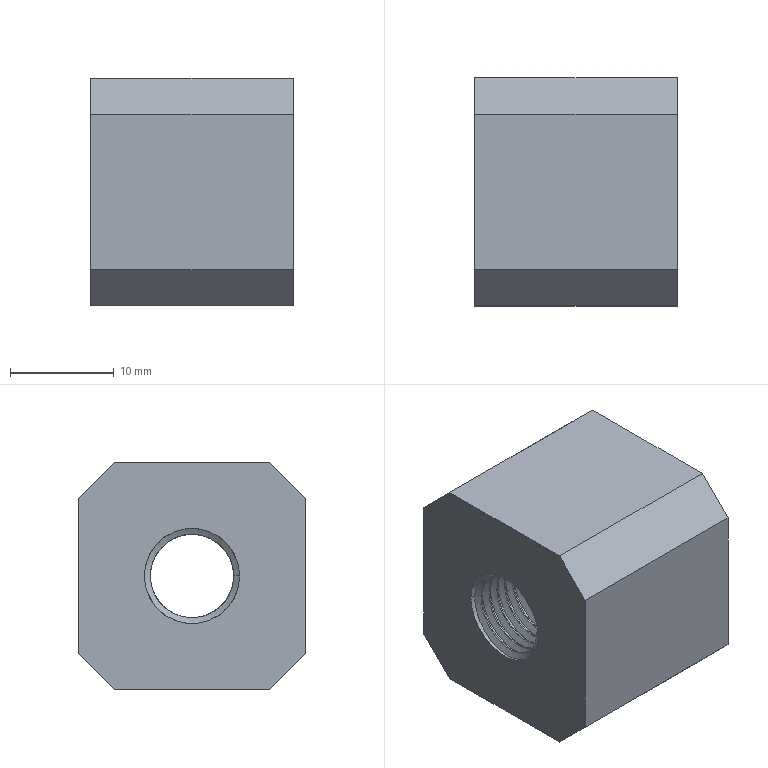Component | SolidWorks | 500CabinetWidthCrossbeamAssembly-1_CrossbeamFixingSleeve-1 | 1 solid | 36 faces | volume 5808 mm3 | cylinder 19 | plane 13 | spline 4 | commonest cylinder face diameters 9.2 x17 17.5 x2 | material Plain Carbon Steel